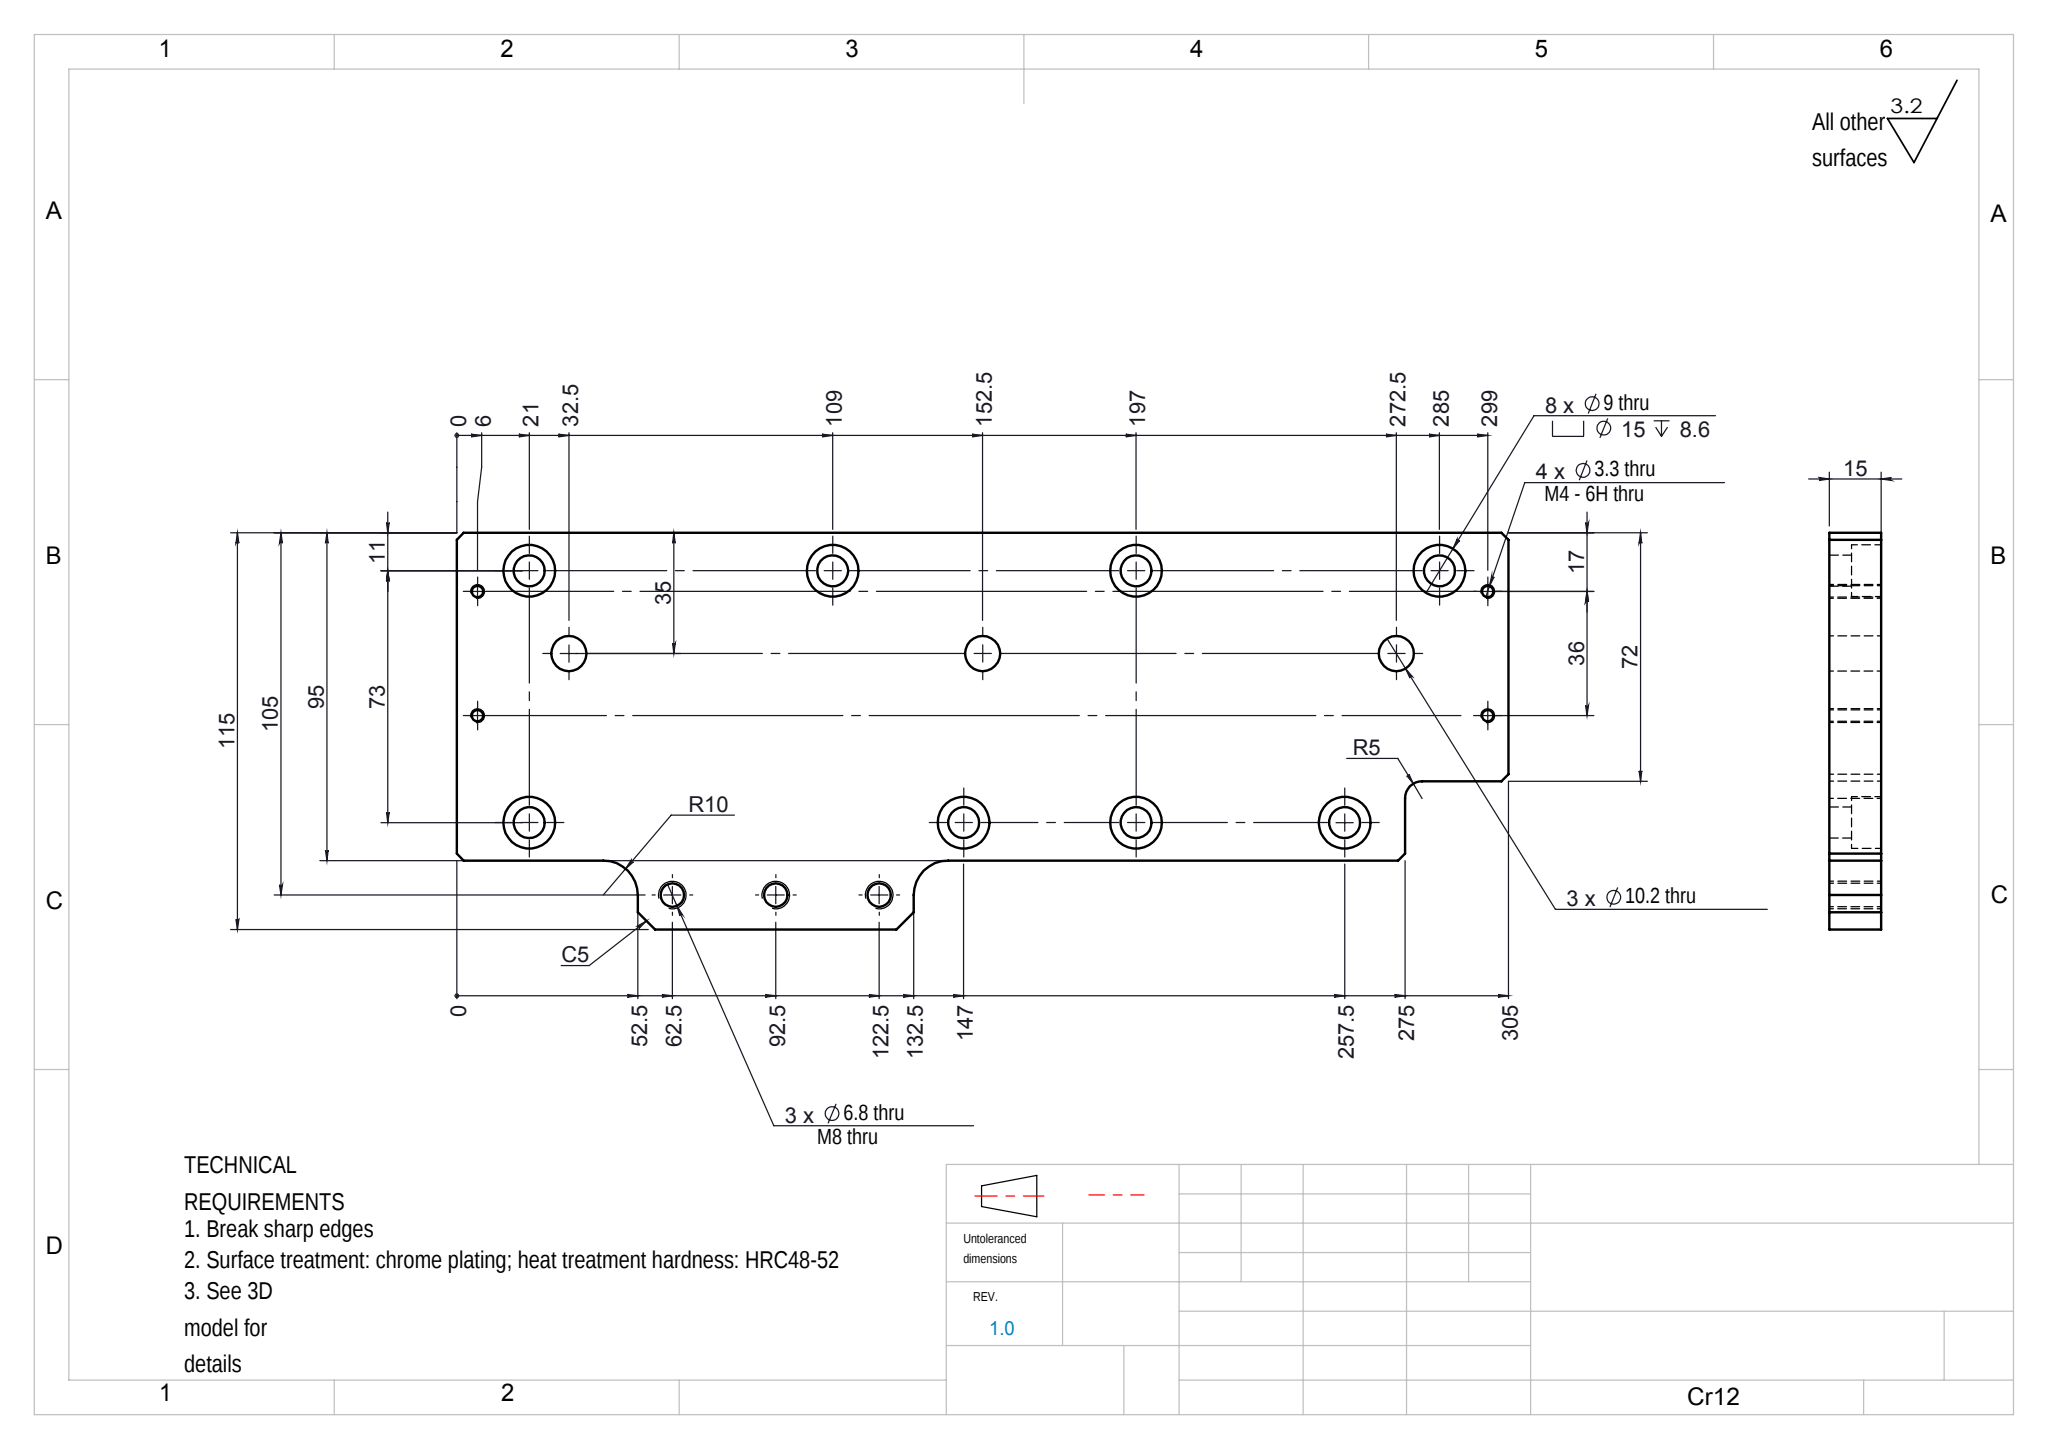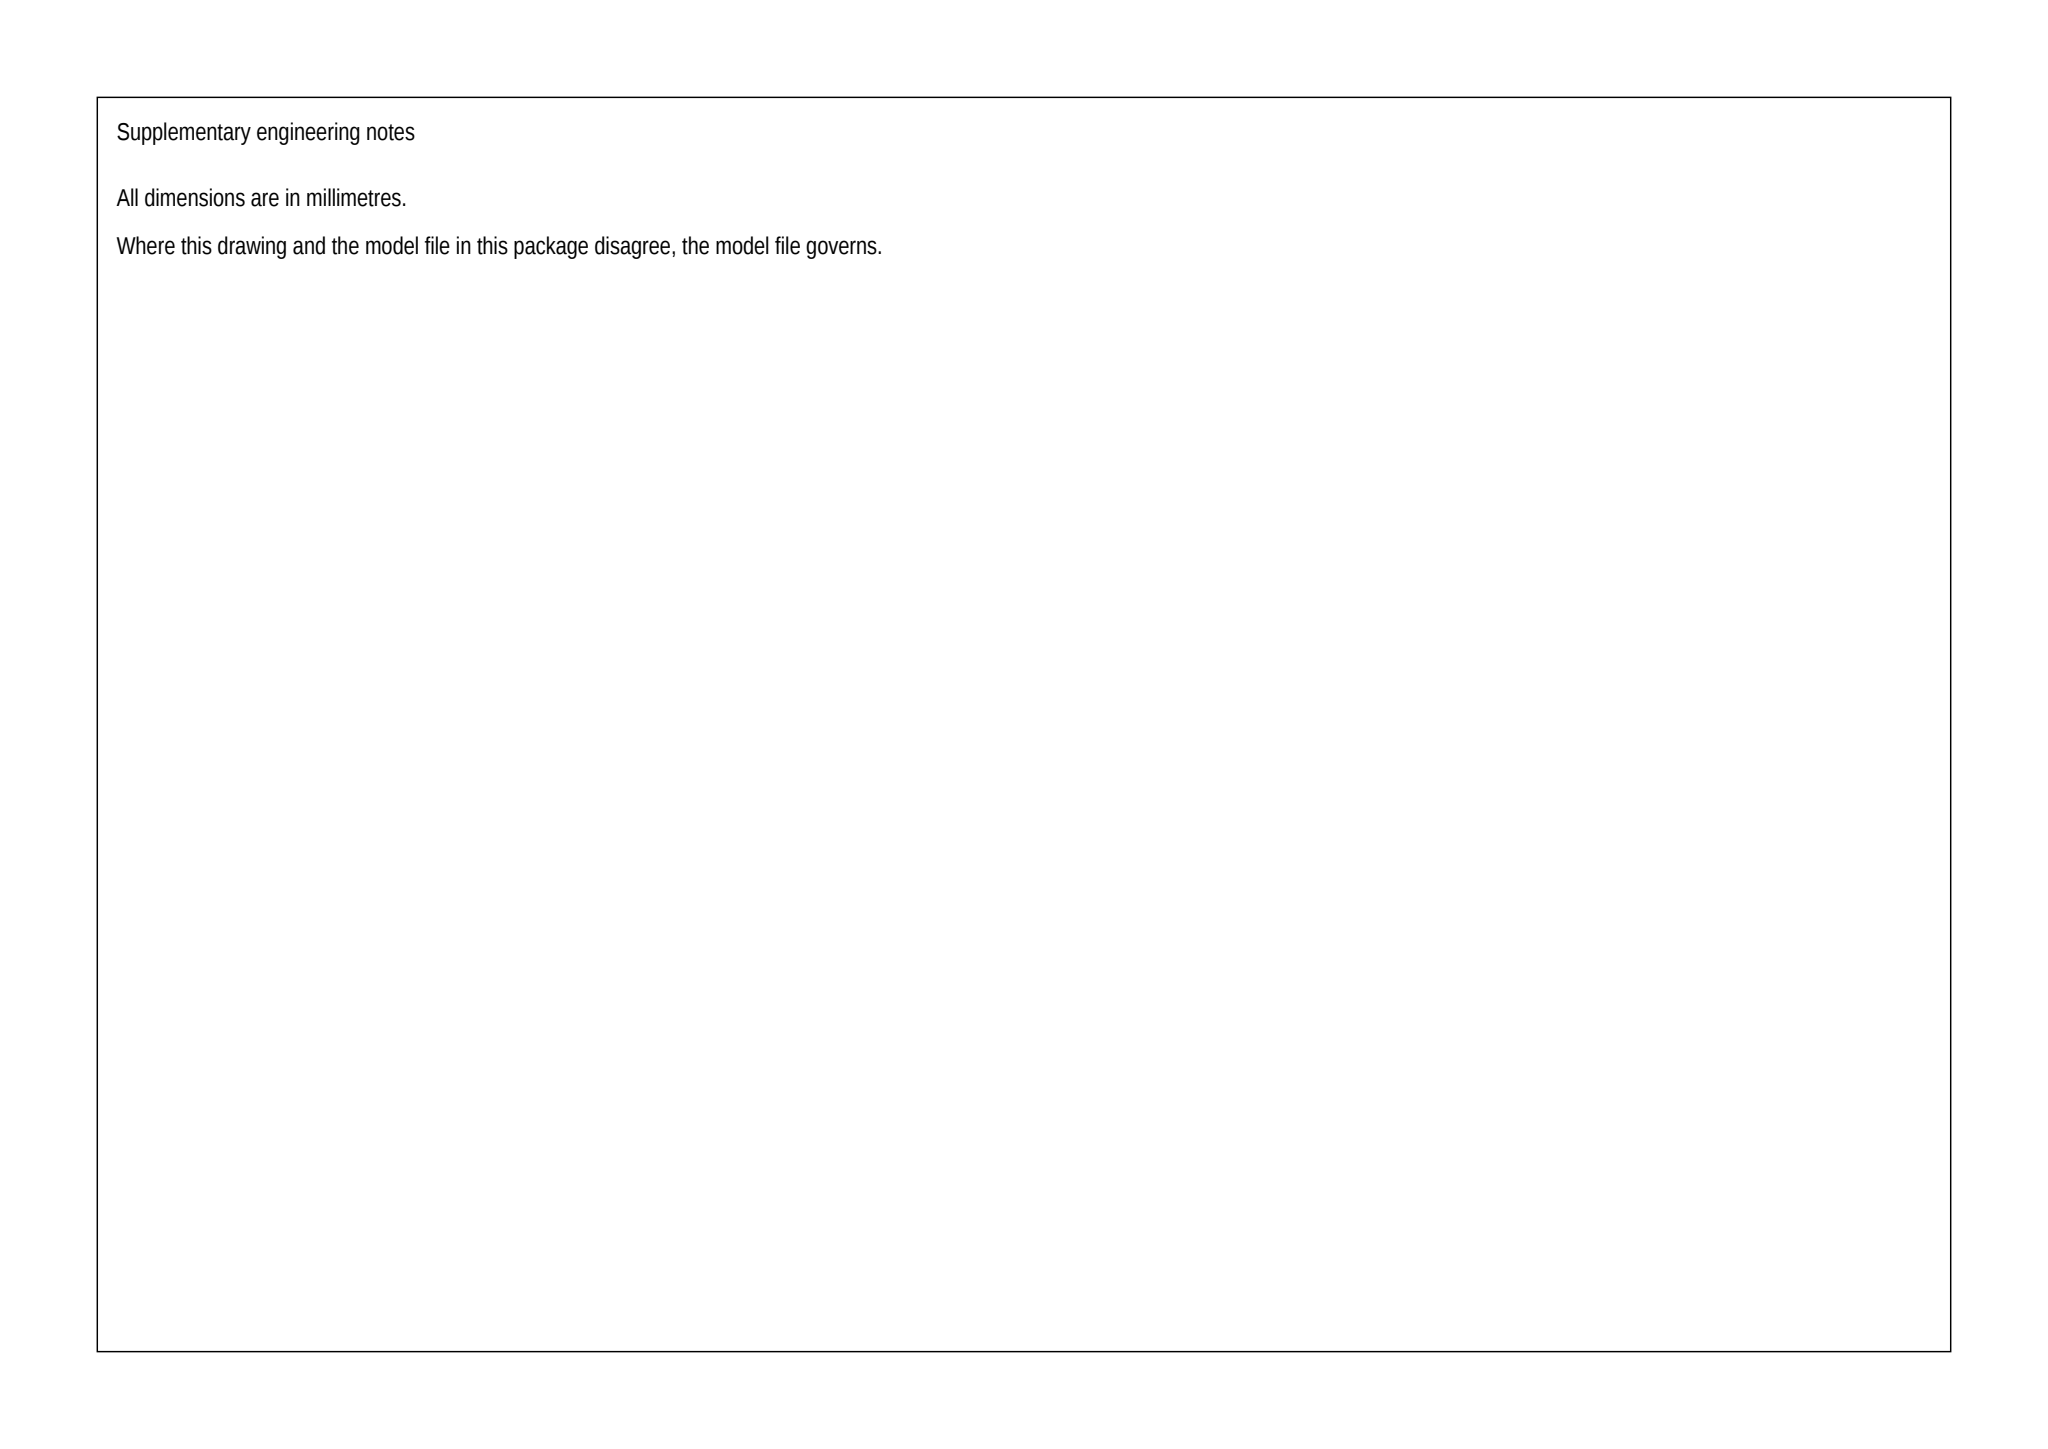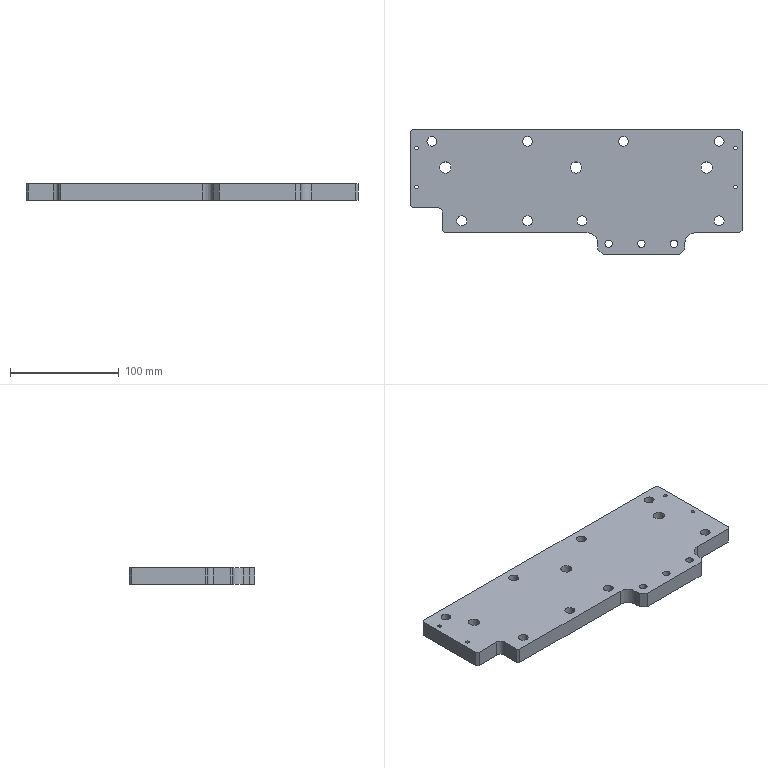Part | SolidWorks | mm | material Cr12 | 1 solid | 82 faces | box 305 x 115 x 15 mm | volume 427235 mm3 | cylinder 55 | plane 27 | commonest cylinder face diameters 15 x16 9 x16 3.3 x8 6.8 x6 10.2 x6 20 x2 10 x1
build123d program:
from build123d import *

# Parameters (mm, degrees)
SKETCH1_W                                       = 305
SKETCH1_H                                       = 95
BOSS_EXTRUDE1_DEPTH                             = 15
F_10_2_10_2_DIAMETER_HOLE1_D                    = 10.2
M8_HEX_SOCKET_HEAD_CAP_SCREW_CBORE1_D           = 9
M8_HEX_SOCKET_HEAD_CAP_SCREW_CBORE1_CBORE_D     = 15
M8_HEX_SOCKET_HEAD_CAP_SCREW_CBORE1_CBORE_DEPTH = 8.6
CHAMFER1_SIZE                                   = 2
M4_TAPPED_HOLE1_D                               = 3.3
SKETCH12_W                                      = 30
SKETCH12_H                                      = 23
CUT_EXTRUDE1_DEPTH                              = 161.429
FILLET1_R                                       = 5
CHAMFER2_SIZE                                   = 2
SKETCH13_W                                      = 80
SKETCH13_H                                      = 20
BOSS_EXTRUDE2_DEPTH                             = 15
M8_TAPPED_HOLE1_D                               = 6.8
FILLET2_R                                       = 10
CHAMFER4_SIZE                                   = 5


with BuildPart() as part:
    # Sketch1 → Boss-Extrude1 (new body)
    with BuildSketch(Plane.XY):
        Rectangle(SKETCH1_W, SKETCH1_H)
    extrude(amount=BOSS_EXTRUDE1_DEPTH)

    # 10.2 _10.2_ Diameter Hole1 (through all)
    with Locations(Plane.XY.offset(15)):
        with Locations((-120, 12.5), (0, 12.5), (120, 12.5)):
            Hole(F_10_2_10_2_DIAMETER_HOLE1_D / 2)

    # M8 Hex Socket Head Cap Screw CBORE1 (through all)
    with Locations(Plane(origin=(0, 0, 0), x_dir=(-1, 0, 0), z_dir=(0, 0, -1))):
        with Locations((132.5, 36.5), (44.5, 36.5), (44.5, -36.5), (-43.5, 36.5), (-5.5, -36.5), (-131.5, 36.5), (-131.5, -36.5), (105, -36.5)):
            CounterBoreHole(M8_HEX_SOCKET_HEAD_CAP_SCREW_CBORE1_D / 2, M8_HEX_SOCKET_HEAD_CAP_SCREW_CBORE1_CBORE_D / 2, M8_HEX_SOCKET_HEAD_CAP_SCREW_CBORE1_CBORE_DEPTH)

    # Chamfer1
    chamfer1_edges = [part.edges().sort_by_distance(p)[0] for p in [
        (152.5, -47.5, 7.5),
        (-152.5, -47.5, 7.5),
        (-152.5, 47.5, 7.5),
        (152.5, 47.5, 7.5),
    ]]
    chamfer(chamfer1_edges, length=CHAMFER1_SIZE)

    # M4 Tapped Hole1 (through all)
    with Locations(Plane(origin=(0, 0, 0), x_dir=(-1, 0, 0), z_dir=(0, 0, -1))):
        with Locations((146.5, -5.5), (146.5, 30.5), (-146.5, -5.5), (-146.5, 30.5)):
            Hole(M4_TAPPED_HOLE1_D / 2)

    # Sketch12 → Cut-Extrude1 (cut, through all)
    with BuildSketch(Plane.XY.offset(15)):
        with Locations((-137.5, -36)):
            Rectangle(SKETCH12_W, SKETCH12_H)
    extrude(amount=-CUT_EXTRUDE1_DEPTH, mode=Mode.SUBTRACT)

    # Fillet1
    fillet1_edges = [part.edges().sort_by_distance(p)[0] for p in [
        (-122.5, -24.5, 7.5),
    ]]
    fillet(fillet1_edges, radius=FILLET1_R)

    # Chamfer2
    chamfer2_edges = [part.edges().sort_by_distance(p)[0] for p in [
        (-152.5, -24.5, 7.5),
        (-122.5, -47.5, 7.5),
    ]]
    chamfer(chamfer2_edges, length=CHAMFER2_SIZE)

    # Sketch13 → Boss-Extrude2 (add)
    with BuildSketch(Plane(origin=(0, 0, 0), x_dir=(-1, 0, 0), z_dir=(0, 0, -1))):
        with Locations((-60, -57.5)):
            Rectangle(SKETCH13_W, SKETCH13_H)
    extrude(amount=-BOSS_EXTRUDE2_DEPTH)

    # M8 Tapped Hole1 (through all)
    with Locations(Plane(origin=(0, 0, 0), x_dir=(-1, 0, 0), z_dir=(0, 0, -1))):
        with Locations((-30, -57.5), (-60, -57.5), (-90, -57.5)):
            Hole(M8_TAPPED_HOLE1_D / 2)

    # Fillet2
    fillet2_edges = [part.edges().sort_by_distance(p)[0] for p in [
        (20, -47.5, 7.5),
        (100, -47.5, 7.5),
    ]]
    fillet(fillet2_edges, radius=FILLET2_R)

    # Chamfer4
    chamfer4_edges = [part.edges().sort_by_distance(p)[0] for p in [
        (20, -67.5, 7.5),
        (100, -67.5, 7.5),
    ]]
    chamfer(chamfer4_edges, length=CHAMFER4_SIZE)


solid = part.part